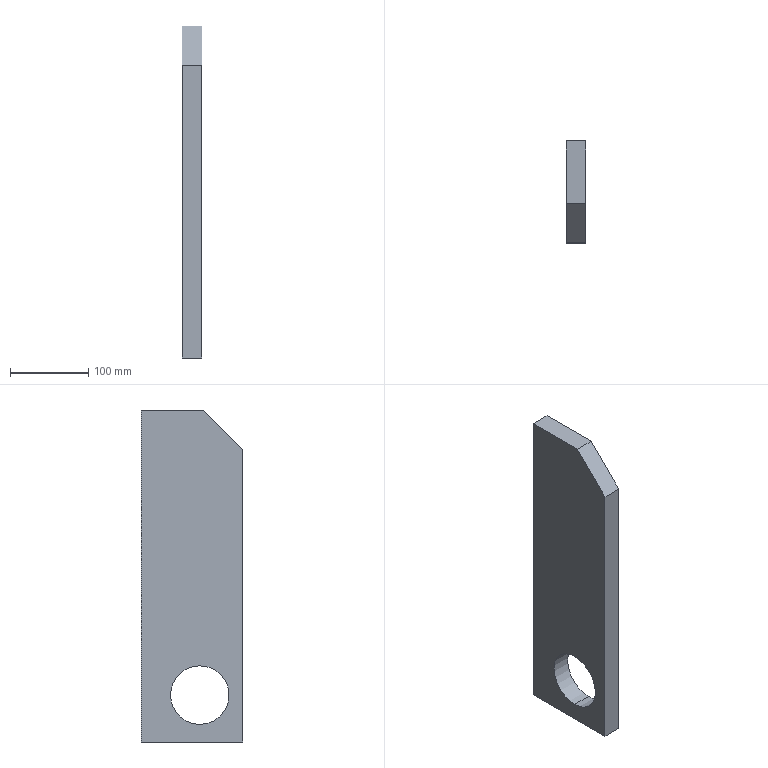Component | SolidWorks | JF21-80.1-1-3(_)-1-SOLID63-1 | 1 solid | 17 faces | box 25 x 130 x 425 mm | volume 1236676 mm3 | plane 7 | cylinder 6 | cone 4 | commonest cylinder face diameters 8.5 x4 75 x2
STEP:
#1=COLOUR_RGB('',0.7922,0.8196,0.9333);
#2=FILL_AREA_STYLE_COLOUR('',#1);
#3=FILL_AREA_STYLE('',(#2));
#4=SURFACE_STYLE_FILL_AREA(#3);
#5=SURFACE_SIDE_STYLE('',(#4));
#6=SURFACE_STYLE_USAGE(.BOTH.,#5);
#7=PRESENTATION_STYLE_ASSIGNMENT((#6));
#8=CARTESIAN_POINT('',(-8.661,13.583,-6.201));
#9=VERTEX_POINT('',#8);
#10=CARTESIAN_POINT('',(-8.661,13.583,-3.248));
#11=VERTEX_POINT('',#10);
#12=CARTESIAN_POINT('',(-8.661,13.583,-4.724));
#13=DIRECTION('',(-1.,0.,0.));
#14=DIRECTION('',(0.,0.,1.));
#15=AXIS2_PLACEMENT_3D('',#12,#13,#14);
#16=CIRCLE('',#15,1.476);
#17=EDGE_CURVE('',#9,#11,#16,.T.);
#18=ORIENTED_EDGE('',*,*,#17,.T.);
#19=CARTESIAN_POINT('',(-7.677,13.583,-3.248));
#20=VERTEX_POINT('',#19);
#21=CARTESIAN_POINT('',(-21.654,13.583,-3.248));
#22=DIRECTION('',(-1.,0.,0.));
#23=VECTOR('',#22,39.37);
#24=LINE('',#21,#23);
#25=EDGE_CURVE('',#20,#11,#24,.T.);
#26=ORIENTED_EDGE('',*,*,#25,.F.);
#27=CARTESIAN_POINT('',(-7.677,13.583,-6.201));
#28=VERTEX_POINT('',#27);
#29=CARTESIAN_POINT('',(-7.677,13.583,-4.724));
#30=DIRECTION('',(1.,0.,-0.));
#31=DIRECTION('',(0.,0.,-1.));
#32=AXIS2_PLACEMENT_3D('',#29,#30,#31);
#33=CIRCLE('',#32,1.476);
#34=EDGE_CURVE('',#20,#28,#33,.T.);
#35=ORIENTED_EDGE('',*,*,#34,.T.);
#36=CARTESIAN_POINT('',(-21.654,13.583,-6.201));
#37=DIRECTION('',(-1.,0.,0.));
#38=VECTOR('',#37,39.37);
#39=LINE('',#36,#38);
#40=EDGE_CURVE('',#28,#9,#39,.T.);
#41=ORIENTED_EDGE('',*,*,#40,.T.);
#42=EDGE_LOOP('',(#18,#26,#35,#41));
#43=FACE_OUTER_BOUND('',#42,.T.);
#44=CARTESIAN_POINT('',(-21.654,13.583,-4.724));
#45=DIRECTION('',(1.,0.,0.));
#46=DIRECTION('',(0.,0.,1.));
#47=AXIS2_PLACEMENT_3D('',#44,#45,#46);
#48=CYLINDRICAL_SURFACE('',#47,1.476);
#49=ADVANCED_FACE('',(#43),#48,.F.);
#50=CARTESIAN_POINT('',(-8.169,15.571,1.703));
#51=VERTEX_POINT('',#50);
#52=CARTESIAN_POINT('',(-8.169,15.571,2.037));
#53=VERTEX_POINT('',#52);
#54=CARTESIAN_POINT('',(-8.169,15.571,1.87));
#55=DIRECTION('',(0.,1.,0.));
#56=DIRECTION('',(0.,0.,1.));
#57=AXIS2_PLACEMENT_3D('',#54,#55,#56);
#58=CIRCLE('',#57,0.1673);
#59=EDGE_CURVE('',#51,#53,#58,.T.);
#60=ORIENTED_EDGE('',*,*,#59,.F.);
#61=CARTESIAN_POINT('',(-8.169,16.535,1.703));
#62=VERTEX_POINT('',#61);
#63=CARTESIAN_POINT('',(-8.169,16.535,1.703));
#64=DIRECTION('',(0.,1.,0.));
#65=VECTOR('',#64,39.37);
#66=LINE('',#63,#65);
#67=EDGE_CURVE('',#51,#62,#66,.T.);
#68=ORIENTED_EDGE('',*,*,#67,.T.);
#69=CARTESIAN_POINT('',(-8.169,16.535,2.037));
#70=VERTEX_POINT('',#69);
#71=CARTESIAN_POINT('',(-8.169,16.535,1.87));
#72=DIRECTION('',(0.,1.,0.));
#73=DIRECTION('',(0.,0.,1.));
#74=AXIS2_PLACEMENT_3D('',#71,#72,#73);
#75=CIRCLE('',#74,0.1673);
#76=EDGE_CURVE('',#62,#70,#75,.T.);
#77=ORIENTED_EDGE('',*,*,#76,.T.);
#78=CARTESIAN_POINT('',(-8.169,16.535,2.037));
#79=DIRECTION('',(0.,1.,0.));
#80=VECTOR('',#79,39.37);
#81=LINE('',#78,#80);
#82=EDGE_CURVE('',#53,#70,#81,.T.);
#83=ORIENTED_EDGE('',*,*,#82,.F.);
#84=EDGE_LOOP('',(#60,#68,#77,#83));
#85=FACE_OUTER_BOUND('',#84,.T.);
#86=CARTESIAN_POINT('',(-8.169,16.535,1.87));
#87=DIRECTION('',(0.,1.,0.));
#88=DIRECTION('',(0.,0.,-1.));
#89=AXIS2_PLACEMENT_3D('',#86,#87,#88);
#90=CYLINDRICAL_SURFACE('',#89,0.1673);
#91=ADVANCED_FACE('',(#85),#90,.F.);
#92=CARTESIAN_POINT('',(-8.169,15.47,1.87));
#93=VERTEX_POINT('',#92);
#94=CARTESIAN_POINT('',(-8.169,15.571,2.037));
#95=DIRECTION('',(0.,0.515,0.8572));
#96=VECTOR('',#95,39.37);
#97=LINE('',#94,#96);
#98=EDGE_CURVE('',#93,#53,#97,.T.);
#99=ORIENTED_EDGE('',*,*,#98,.F.);
#100=CARTESIAN_POINT('',(-8.169,15.571,1.703));
#101=DIRECTION('',(0.,0.515,-0.8572));
#102=VECTOR('',#101,39.37);
#103=LINE('',#100,#102);
#104=EDGE_CURVE('',#93,#51,#103,.T.);
#105=ORIENTED_EDGE('',*,*,#104,.T.);
#106=ORIENTED_EDGE('',*,*,#59,.T.);
#107=EDGE_LOOP('',(#99,#105,#106));
#108=FACE_OUTER_BOUND('',#107,.T.);
#109=CARTESIAN_POINT('',(-8.169,15.571,1.87));
#110=DIRECTION('',(0.,1.,0.));
#111=DIRECTION('',(0.,0.,-1.));
#112=AXIS2_PLACEMENT_3D('',#109,#110,#111);
#113=CONICAL_SURFACE('',#112,0.1673,1.03);
#114=ADVANCED_FACE('',(#108),#113,.F.);
#115=CARTESIAN_POINT('',(-8.169,15.571,8.199));
#116=VERTEX_POINT('',#115);
#117=CARTESIAN_POINT('',(-8.169,15.571,8.533));
#118=VERTEX_POINT('',#117);
#119=CARTESIAN_POINT('',(-8.169,15.571,8.366));
#120=DIRECTION('',(0.,1.,0.));
#121=DIRECTION('',(0.,0.,1.));
#122=AXIS2_PLACEMENT_3D('',#119,#120,#121);
#123=CIRCLE('',#122,0.1673);
#124=EDGE_CURVE('',#116,#118,#123,.T.);
#125=ORIENTED_EDGE('',*,*,#124,.F.);
#126=CARTESIAN_POINT('',(-8.169,16.535,8.199));
#127=VERTEX_POINT('',#126);
#128=CARTESIAN_POINT('',(-8.169,16.535,8.199));
#129=DIRECTION('',(0.,1.,0.));
#130=VECTOR('',#129,39.37);
#131=LINE('',#128,#130);
#132=EDGE_CURVE('',#116,#127,#131,.T.);
#133=ORIENTED_EDGE('',*,*,#132,.T.);
#134=CARTESIAN_POINT('',(-8.169,16.535,8.533));
#135=VERTEX_POINT('',#134);
#136=CARTESIAN_POINT('',(-8.169,16.535,8.366));
#137=DIRECTION('',(0.,1.,0.));
#138=DIRECTION('',(0.,0.,1.));
#139=AXIS2_PLACEMENT_3D('',#136,#137,#138);
#140=CIRCLE('',#139,0.1673);
#141=EDGE_CURVE('',#127,#135,#140,.T.);
#142=ORIENTED_EDGE('',*,*,#141,.T.);
#143=CARTESIAN_POINT('',(-8.169,16.535,8.533));
#144=DIRECTION('',(0.,1.,0.));
#145=VECTOR('',#144,39.37);
#146=LINE('',#143,#145);
#147=EDGE_CURVE('',#118,#135,#146,.T.);
#148=ORIENTED_EDGE('',*,*,#147,.F.);
#149=EDGE_LOOP('',(#125,#133,#142,#148));
#150=FACE_OUTER_BOUND('',#149,.T.);
#151=CARTESIAN_POINT('',(-8.169,16.535,8.366));
#152=DIRECTION('',(0.,1.,0.));
#153=DIRECTION('',(0.,0.,-1.));
#154=AXIS2_PLACEMENT_3D('',#151,#152,#153);
#155=CYLINDRICAL_SURFACE('',#154,0.1673);
#156=ADVANCED_FACE('',(#150),#155,.F.);
#157=CARTESIAN_POINT('',(-8.169,15.47,8.366));
#158=VERTEX_POINT('',#157);
#159=CARTESIAN_POINT('',(-8.169,15.571,8.533));
#160=DIRECTION('',(0.,0.515,0.8572));
#161=VECTOR('',#160,39.37);
#162=LINE('',#159,#161);
#163=EDGE_CURVE('',#158,#118,#162,.T.);
#164=ORIENTED_EDGE('',*,*,#163,.F.);
#165=CARTESIAN_POINT('',(-8.169,15.571,8.199));
#166=DIRECTION('',(0.,0.515,-0.8572));
#167=VECTOR('',#166,39.37);
#168=LINE('',#165,#167);
#169=EDGE_CURVE('',#158,#116,#168,.T.);
#170=ORIENTED_EDGE('',*,*,#169,.T.);
#171=ORIENTED_EDGE('',*,*,#124,.T.);
#172=EDGE_LOOP('',(#164,#170,#171));
#173=FACE_OUTER_BOUND('',#172,.T.);
#174=CARTESIAN_POINT('',(-8.169,15.571,8.366));
#175=DIRECTION('',(0.,1.,0.));
#176=DIRECTION('',(0.,0.,-1.));
#177=AXIS2_PLACEMENT_3D('',#174,#175,#176);
#178=CONICAL_SURFACE('',#177,0.1673,1.03);
#179=ADVANCED_FACE('',(#173),#178,.F.);
#180=ORIENTED_EDGE('',*,*,#17,.F.);
#181=CARTESIAN_POINT('',(-8.661,13.583,-4.724));
#182=DIRECTION('',(-1.,0.,0.));
#183=DIRECTION('',(0.,0.,1.));
#184=AXIS2_PLACEMENT_3D('',#181,#182,#183);
#185=CIRCLE('',#184,1.476);
#186=EDGE_CURVE('',#11,#9,#185,.T.);
#187=ORIENTED_EDGE('',*,*,#186,.F.);
#188=EDGE_LOOP('',(#180,#187));
#189=FACE_BOUND('',#188,.T.);
#190=CARTESIAN_POINT('',(-8.661,11.417,-7.087));
#191=VERTEX_POINT('',#190);
#192=CARTESIAN_POINT('',(-8.661,11.417,7.677));
#193=VERTEX_POINT('',#192);
#194=CARTESIAN_POINT('',(-8.661,11.417,-7.087));
#195=DIRECTION('',(0.,0.,1.));
#196=VECTOR('',#195,39.37);
#197=LINE('',#194,#196);
#198=EDGE_CURVE('',#191,#193,#197,.T.);
#199=ORIENTED_EDGE('',*,*,#198,.T.);
#200=CARTESIAN_POINT('',(-8.661,13.386,9.646));
#201=VERTEX_POINT('',#200);
#202=CARTESIAN_POINT('',(-8.661,4.035,0.2953));
#203=DIRECTION('',(0.,0.7071,0.7071));
#204=VECTOR('',#203,39.37);
#205=LINE('',#202,#204);
#206=EDGE_CURVE('',#193,#201,#205,.T.);
#207=ORIENTED_EDGE('',*,*,#206,.T.);
#208=CARTESIAN_POINT('',(-8.661,16.535,9.646));
#209=VERTEX_POINT('',#208);
#210=CARTESIAN_POINT('',(-8.661,11.417,9.646));
#211=DIRECTION('',(0.,1.,0.));
#212=VECTOR('',#211,39.37);
#213=LINE('',#210,#212);
#214=EDGE_CURVE('',#201,#209,#213,.T.);
#215=ORIENTED_EDGE('',*,*,#214,.T.);
#216=CARTESIAN_POINT('',(-8.661,16.535,-7.087));
#217=VERTEX_POINT('',#216);
#218=CARTESIAN_POINT('',(-8.661,16.535,-7.087));
#219=DIRECTION('',(0.,0.,1.));
#220=VECTOR('',#219,39.37);
#221=LINE('',#218,#220);
#222=EDGE_CURVE('',#217,#209,#221,.T.);
#223=ORIENTED_EDGE('',*,*,#222,.F.);
#224=CARTESIAN_POINT('',(-8.661,11.417,-7.087));
#225=DIRECTION('',(0.,1.,0.));
#226=VECTOR('',#225,39.37);
#227=LINE('',#224,#226);
#228=EDGE_CURVE('',#191,#217,#227,.T.);
#229=ORIENTED_EDGE('',*,*,#228,.F.);
#230=EDGE_LOOP('',(#199,#207,#215,#223,#229));
#231=FACE_OUTER_BOUND('',#230,.T.);
#232=CARTESIAN_POINT('',(-8.661,11.417,-7.087));
#233=DIRECTION('',(-1.,0.,0.));
#234=DIRECTION('',(-0.,0.,-1.));
#235=AXIS2_PLACEMENT_3D('',#232,#233,#234);
#236=PLANE('',#235);
#237=ADVANCED_FACE('',(#189,#231),#236,.T.);
#238=CARTESIAN_POINT('',(-7.677,16.535,-7.087));
#239=VERTEX_POINT('',#238);
#240=CARTESIAN_POINT('',(-8.661,16.535,-7.087));
#241=DIRECTION('',(-1.,0.,0.));
#242=VECTOR('',#241,39.37);
#243=LINE('',#240,#242);
#244=EDGE_CURVE('',#239,#217,#243,.T.);
#245=ORIENTED_EDGE('',*,*,#244,.F.);
#246=CARTESIAN_POINT('',(-7.677,11.417,-7.087));
#247=VERTEX_POINT('',#246);
#248=CARTESIAN_POINT('',(-7.677,11.417,-7.087));
#249=DIRECTION('',(0.,1.,0.));
#250=VECTOR('',#249,39.37);
#251=LINE('',#248,#250);
#252=EDGE_CURVE('',#247,#239,#251,.T.);
#253=ORIENTED_EDGE('',*,*,#252,.F.);
#254=CARTESIAN_POINT('',(-8.661,11.417,-7.087));
#255=DIRECTION('',(-1.,0.,0.));
#256=VECTOR('',#255,39.37);
#257=LINE('',#254,#256);
#258=EDGE_CURVE('',#247,#191,#257,.T.);
#259=ORIENTED_EDGE('',*,*,#258,.T.);
#260=ORIENTED_EDGE('',*,*,#228,.T.);
#261=EDGE_LOOP('',(#245,#253,#259,#260));
#262=FACE_OUTER_BOUND('',#261,.T.);
#263=CARTESIAN_POINT('',(-8.661,11.417,-7.087));
#264=DIRECTION('',(0.,0.,-1.));
#265=DIRECTION('',(1.,0.,0.));
#266=AXIS2_PLACEMENT_3D('',#263,#264,#265);
#267=PLANE('',#266);
#268=ADVANCED_FACE('',(#262),#267,.T.);
#269=CARTESIAN_POINT('',(-7.677,13.583,-4.724));
#270=DIRECTION('',(1.,0.,-0.));
#271=DIRECTION('',(0.,0.,-1.));
#272=AXIS2_PLACEMENT_3D('',#269,#270,#271);
#273=CIRCLE('',#272,1.476);
#274=EDGE_CURVE('',#28,#20,#273,.T.);
#275=ORIENTED_EDGE('',*,*,#274,.F.);
#276=ORIENTED_EDGE('',*,*,#34,.F.);
#277=EDGE_LOOP('',(#275,#276));
#278=FACE_BOUND('',#277,.T.);
#279=CARTESIAN_POINT('',(-7.677,13.386,9.646));
#280=VERTEX_POINT('',#279);
#281=CARTESIAN_POINT('',(-7.677,16.535,9.646));
#282=VERTEX_POINT('',#281);
#283=CARTESIAN_POINT('',(-7.677,11.417,9.646));
#284=DIRECTION('',(0.,1.,0.));
#285=VECTOR('',#284,39.37);
#286=LINE('',#283,#285);
#287=EDGE_CURVE('',#280,#282,#286,.T.);
#288=ORIENTED_EDGE('',*,*,#287,.F.);
#289=CARTESIAN_POINT('',(-7.677,11.417,7.677));
#290=VERTEX_POINT('',#289);
#291=CARTESIAN_POINT('',(-7.677,4.035,0.2953));
#292=DIRECTION('',(-0.,-0.7071,-0.7071));
#293=VECTOR('',#292,39.37);
#294=LINE('',#291,#293);
#295=EDGE_CURVE('',#280,#290,#294,.T.);
#296=ORIENTED_EDGE('',*,*,#295,.T.);
#297=CARTESIAN_POINT('',(-7.677,11.417,-7.087));
#298=DIRECTION('',(-0.,0.,-1.));
#299=VECTOR('',#298,39.37);
#300=LINE('',#297,#299);
#301=EDGE_CURVE('',#290,#247,#300,.T.);
#302=ORIENTED_EDGE('',*,*,#301,.T.);
#303=ORIENTED_EDGE('',*,*,#252,.T.);
#304=CARTESIAN_POINT('',(-7.677,16.535,-7.087));
#305=DIRECTION('',(-0.,0.,-1.));
#306=VECTOR('',#305,39.37);
#307=LINE('',#304,#306);
#308=EDGE_CURVE('',#282,#239,#307,.T.);
#309=ORIENTED_EDGE('',*,*,#308,.F.);
#310=EDGE_LOOP('',(#288,#296,#302,#303,#309));
#311=FACE_OUTER_BOUND('',#310,.T.);
#312=CARTESIAN_POINT('',(-7.677,11.417,-7.087));
#313=DIRECTION('',(1.,0.,-0.));
#314=DIRECTION('',(0.,0.,1.));
#315=AXIS2_PLACEMENT_3D('',#312,#313,#314);
#316=PLANE('',#315);
#317=ADVANCED_FACE('',(#278,#311),#316,.T.);
#318=ORIENTED_EDGE('',*,*,#214,.F.);
#319=CARTESIAN_POINT('',(-7.677,13.386,9.646));
#320=DIRECTION('',(1.,0.,0.));
#321=VECTOR('',#320,39.37);
#322=LINE('',#319,#321);
#323=EDGE_CURVE('',#201,#280,#322,.T.);
#324=ORIENTED_EDGE('',*,*,#323,.T.);
#325=ORIENTED_EDGE('',*,*,#287,.T.);
#326=CARTESIAN_POINT('',(-8.661,16.535,9.646));
#327=DIRECTION('',(1.,0.,0.));
#328=VECTOR('',#327,39.37);
#329=LINE('',#326,#328);
#330=EDGE_CURVE('',#209,#282,#329,.T.);
#331=ORIENTED_EDGE('',*,*,#330,.F.);
#332=EDGE_LOOP('',(#318,#324,#325,#331));
#333=FACE_OUTER_BOUND('',#332,.T.);
#334=CARTESIAN_POINT('',(-8.661,11.417,9.646));
#335=DIRECTION('',(0.,0.,1.));
#336=DIRECTION('',(-1.,0.,0.));
#337=AXIS2_PLACEMENT_3D('',#334,#335,#336);
#338=PLANE('',#337);
#339=ADVANCED_FACE('',(#333),#338,.T.);
#340=ORIENTED_EDGE('',*,*,#301,.F.);
#341=CARTESIAN_POINT('',(-8.661,11.417,7.677));
#342=DIRECTION('',(-1.,0.,0.));
#343=VECTOR('',#342,39.37);
#344=LINE('',#341,#343);
#345=EDGE_CURVE('',#290,#193,#344,.T.);
#346=ORIENTED_EDGE('',*,*,#345,.T.);
#347=ORIENTED_EDGE('',*,*,#198,.F.);
#348=ORIENTED_EDGE('',*,*,#258,.F.);
#349=EDGE_LOOP('',(#340,#346,#347,#348));
#350=FACE_OUTER_BOUND('',#349,.T.);
#351=CARTESIAN_POINT('',(-8.661,11.417,9.646));
#352=DIRECTION('',(0.,1.,0.));
#353=DIRECTION('',(0.,0.,-1.));
#354=AXIS2_PLACEMENT_3D('',#351,#352,#353);
#355=PLANE('',#354);
#356=ADVANCED_FACE('',(#350),#355,.F.);
#357=CARTESIAN_POINT('',(-8.169,16.535,1.87));
#358=DIRECTION('',(0.,1.,0.));
#359=DIRECTION('',(0.,0.,1.));
#360=AXIS2_PLACEMENT_3D('',#357,#358,#359);
#361=CIRCLE('',#360,0.1673);
#362=EDGE_CURVE('',#70,#62,#361,.T.);
#363=ORIENTED_EDGE('',*,*,#362,.F.);
#364=ORIENTED_EDGE('',*,*,#76,.F.);
#365=EDGE_LOOP('',(#363,#364));
#366=FACE_BOUND('',#365,.T.);
#367=CARTESIAN_POINT('',(-8.169,16.535,8.366));
#368=DIRECTION('',(0.,1.,0.));
#369=DIRECTION('',(0.,0.,1.));
#370=AXIS2_PLACEMENT_3D('',#367,#368,#369);
#371=CIRCLE('',#370,0.1673);
#372=EDGE_CURVE('',#135,#127,#371,.T.);
#373=ORIENTED_EDGE('',*,*,#372,.F.);
#374=ORIENTED_EDGE('',*,*,#141,.F.);
#375=EDGE_LOOP('',(#373,#374));
#376=FACE_BOUND('',#375,.T.);
#377=ORIENTED_EDGE('',*,*,#222,.T.);
#378=ORIENTED_EDGE('',*,*,#330,.T.);
#379=ORIENTED_EDGE('',*,*,#308,.T.);
#380=ORIENTED_EDGE('',*,*,#244,.T.);
#381=EDGE_LOOP('',(#377,#378,#379,#380));
#382=FACE_OUTER_BOUND('',#381,.T.);
#383=CARTESIAN_POINT('',(-8.661,16.535,9.646));
#384=DIRECTION('',(0.,1.,0.));
#385=DIRECTION('',(0.,0.,-1.));
#386=AXIS2_PLACEMENT_3D('',#383,#384,#385);
#387=PLANE('',#386);
#388=ADVANCED_FACE('',(#366,#376,#382),#387,.T.);
#389=ORIENTED_EDGE('',*,*,#206,.F.);
#390=ORIENTED_EDGE('',*,*,#345,.F.);
#391=ORIENTED_EDGE('',*,*,#295,.F.);
#392=ORIENTED_EDGE('',*,*,#323,.F.);
#393=EDGE_LOOP('',(#389,#390,#391,#392));
#394=FACE_OUTER_BOUND('',#393,.T.);
#395=CARTESIAN_POINT('',(-8.661,13.386,9.646));
#396=DIRECTION('',(0.,-0.7071,0.7071));
#397=DIRECTION('',(0.,0.7071,0.7071));
#398=AXIS2_PLACEMENT_3D('',#395,#396,#397);
#399=PLANE('',#398);
#400=ADVANCED_FACE('',(#394),#399,.T.);
#401=ORIENTED_EDGE('',*,*,#169,.F.);
#402=ORIENTED_EDGE('',*,*,#163,.T.);
#403=CARTESIAN_POINT('',(-8.169,15.571,8.366));
#404=DIRECTION('',(0.,1.,0.));
#405=DIRECTION('',(0.,0.,1.));
#406=AXIS2_PLACEMENT_3D('',#403,#404,#405);
#407=CIRCLE('',#406,0.1673);
#408=EDGE_CURVE('',#118,#116,#407,.T.);
#409=ORIENTED_EDGE('',*,*,#408,.T.);
#410=EDGE_LOOP('',(#401,#402,#409));
#411=FACE_OUTER_BOUND('',#410,.T.);
#412=CARTESIAN_POINT('',(-8.169,15.571,8.366));
#413=DIRECTION('',(0.,1.,0.));
#414=DIRECTION('',(0.,0.,-1.));
#415=AXIS2_PLACEMENT_3D('',#412,#413,#414);
#416=CONICAL_SURFACE('',#415,0.1673,1.03);
#417=ADVANCED_FACE('',(#411),#416,.F.);
#418=ORIENTED_EDGE('',*,*,#132,.F.);
#419=ORIENTED_EDGE('',*,*,#408,.F.);
#420=ORIENTED_EDGE('',*,*,#147,.T.);
#421=ORIENTED_EDGE('',*,*,#372,.T.);
#422=EDGE_LOOP('',(#418,#419,#420,#421));
#423=FACE_OUTER_BOUND('',#422,.T.);
#424=CARTESIAN_POINT('',(-8.169,16.535,8.366));
#425=DIRECTION('',(0.,1.,0.));
#426=DIRECTION('',(0.,0.,-1.));
#427=AXIS2_PLACEMENT_3D('',#424,#425,#426);
#428=CYLINDRICAL_SURFACE('',#427,0.1673);
#429=ADVANCED_FACE('',(#423),#428,.F.);
#430=ORIENTED_EDGE('',*,*,#104,.F.);
#431=ORIENTED_EDGE('',*,*,#98,.T.);
#432=CARTESIAN_POINT('',(-8.169,15.571,1.87));
#433=DIRECTION('',(0.,1.,0.));
#434=DIRECTION('',(0.,0.,1.));
#435=AXIS2_PLACEMENT_3D('',#432,#433,#434);
#436=CIRCLE('',#435,0.1673);
#437=EDGE_CURVE('',#53,#51,#436,.T.);
#438=ORIENTED_EDGE('',*,*,#437,.T.);
#439=EDGE_LOOP('',(#430,#431,#438));
#440=FACE_OUTER_BOUND('',#439,.T.);
#441=CARTESIAN_POINT('',(-8.169,15.571,1.87));
#442=DIRECTION('',(0.,1.,0.));
#443=DIRECTION('',(0.,0.,-1.));
#444=AXIS2_PLACEMENT_3D('',#441,#442,#443);
#445=CONICAL_SURFACE('',#444,0.1673,1.03);
#446=ADVANCED_FACE('',(#440),#445,.F.);
#447=ORIENTED_EDGE('',*,*,#67,.F.);
#448=ORIENTED_EDGE('',*,*,#437,.F.);
#449=ORIENTED_EDGE('',*,*,#82,.T.);
#450=ORIENTED_EDGE('',*,*,#362,.T.);
#451=EDGE_LOOP('',(#447,#448,#449,#450));
#452=FACE_OUTER_BOUND('',#451,.T.);
#453=CARTESIAN_POINT('',(-8.169,16.535,1.87));
#454=DIRECTION('',(0.,1.,0.));
#455=DIRECTION('',(0.,0.,-1.));
#456=AXIS2_PLACEMENT_3D('',#453,#454,#455);
#457=CYLINDRICAL_SURFACE('',#456,0.1673);
#458=ADVANCED_FACE('',(#452),#457,.F.);
#459=ORIENTED_EDGE('',*,*,#25,.T.);
#460=ORIENTED_EDGE('',*,*,#186,.T.);
#461=ORIENTED_EDGE('',*,*,#40,.F.);
#462=ORIENTED_EDGE('',*,*,#274,.T.);
#463=EDGE_LOOP('',(#459,#460,#461,#462));
#464=FACE_OUTER_BOUND('',#463,.T.);
#465=CARTESIAN_POINT('',(-21.654,13.583,-4.724));
#466=DIRECTION('',(1.,0.,0.));
#467=DIRECTION('',(0.,0.,1.));
#468=AXIS2_PLACEMENT_3D('',#465,#466,#467);
#469=CYLINDRICAL_SURFACE('',#468,1.476);
#470=ADVANCED_FACE('',(#464),#469,.F.);
#471=CLOSED_SHELL('',(#49,#91,#114,#156,#179,#237,#268,#317,#339,#356,#388,#400,#417,#429,#446,#458,#470));
#472=MANIFOLD_SOLID_BREP('',#471);
#473=STYLED_ITEM('',(#7),#472);
#474=(LENGTH_UNIT()NAMED_UNIT(*)SI_UNIT($,.METRE.));
#475=LENGTH_MEASURE_WITH_UNIT(LENGTH_MEASURE(0.0254),#474);
#476=DIMENSIONAL_EXPONENTS(1.,0.,0.,0.,0.,0.,0.);
#477=(CONVERSION_BASED_UNIT('',#475)LENGTH_UNIT()NAMED_UNIT(#476));
#478=UNCERTAINTY_MEASURE_WITH_UNIT(LENGTH_MEASURE(0.00001),#477,'','');
#479=(NAMED_UNIT(*)PLANE_ANGLE_UNIT()SI_UNIT($,.RADIAN.));
#480=(NAMED_UNIT(*)SI_UNIT($,.STERADIAN.)SOLID_ANGLE_UNIT());
#481=(GEOMETRIC_REPRESENTATION_CONTEXT(3)GLOBAL_UNCERTAINTY_ASSIGNED_CONTEXT((#478))GLOBAL_UNIT_ASSIGNED_CONTEXT((#477,#479,#480))REPRESENTATION_CONTEXT('',''));
#482=MECHANICAL_DESIGN_GEOMETRIC_PRESENTATION_REPRESENTATION('',(#473),#481);
#483=CARTESIAN_POINT('',(0.,0.,0.));
#484=DIRECTION('',(0.,0.,1.));
#485=DIRECTION('',(1.,0.,0.));
#486=AXIS2_PLACEMENT_3D('',#483,#484,#485);
#487=(LENGTH_UNIT()NAMED_UNIT(*)SI_UNIT($,.METRE.));
#488=LENGTH_MEASURE_WITH_UNIT(LENGTH_MEASURE(0.0254),#487);
#489=DIMENSIONAL_EXPONENTS(1.,0.,0.,0.,0.,0.,0.);
#490=(CONVERSION_BASED_UNIT('',#488)LENGTH_UNIT()NAMED_UNIT(#489));
#491=UNCERTAINTY_MEASURE_WITH_UNIT(LENGTH_MEASURE(0.00001),#490,'','');
#492=(NAMED_UNIT(*)PLANE_ANGLE_UNIT()SI_UNIT($,.RADIAN.));
#493=(NAMED_UNIT(*)SI_UNIT($,.STERADIAN.)SOLID_ANGLE_UNIT());
#494=(GEOMETRIC_REPRESENTATION_CONTEXT(3)GLOBAL_UNCERTAINTY_ASSIGNED_CONTEXT((#491))GLOBAL_UNIT_ASSIGNED_CONTEXT((#490,#492,#493))REPRESENTATION_CONTEXT('',''));
#495=ADVANCED_BREP_SHAPE_REPRESENTATION('',(#472,#486),#494);
#496=PRESENTATION_LAYER_ASSIGNMENT('','',(#473));